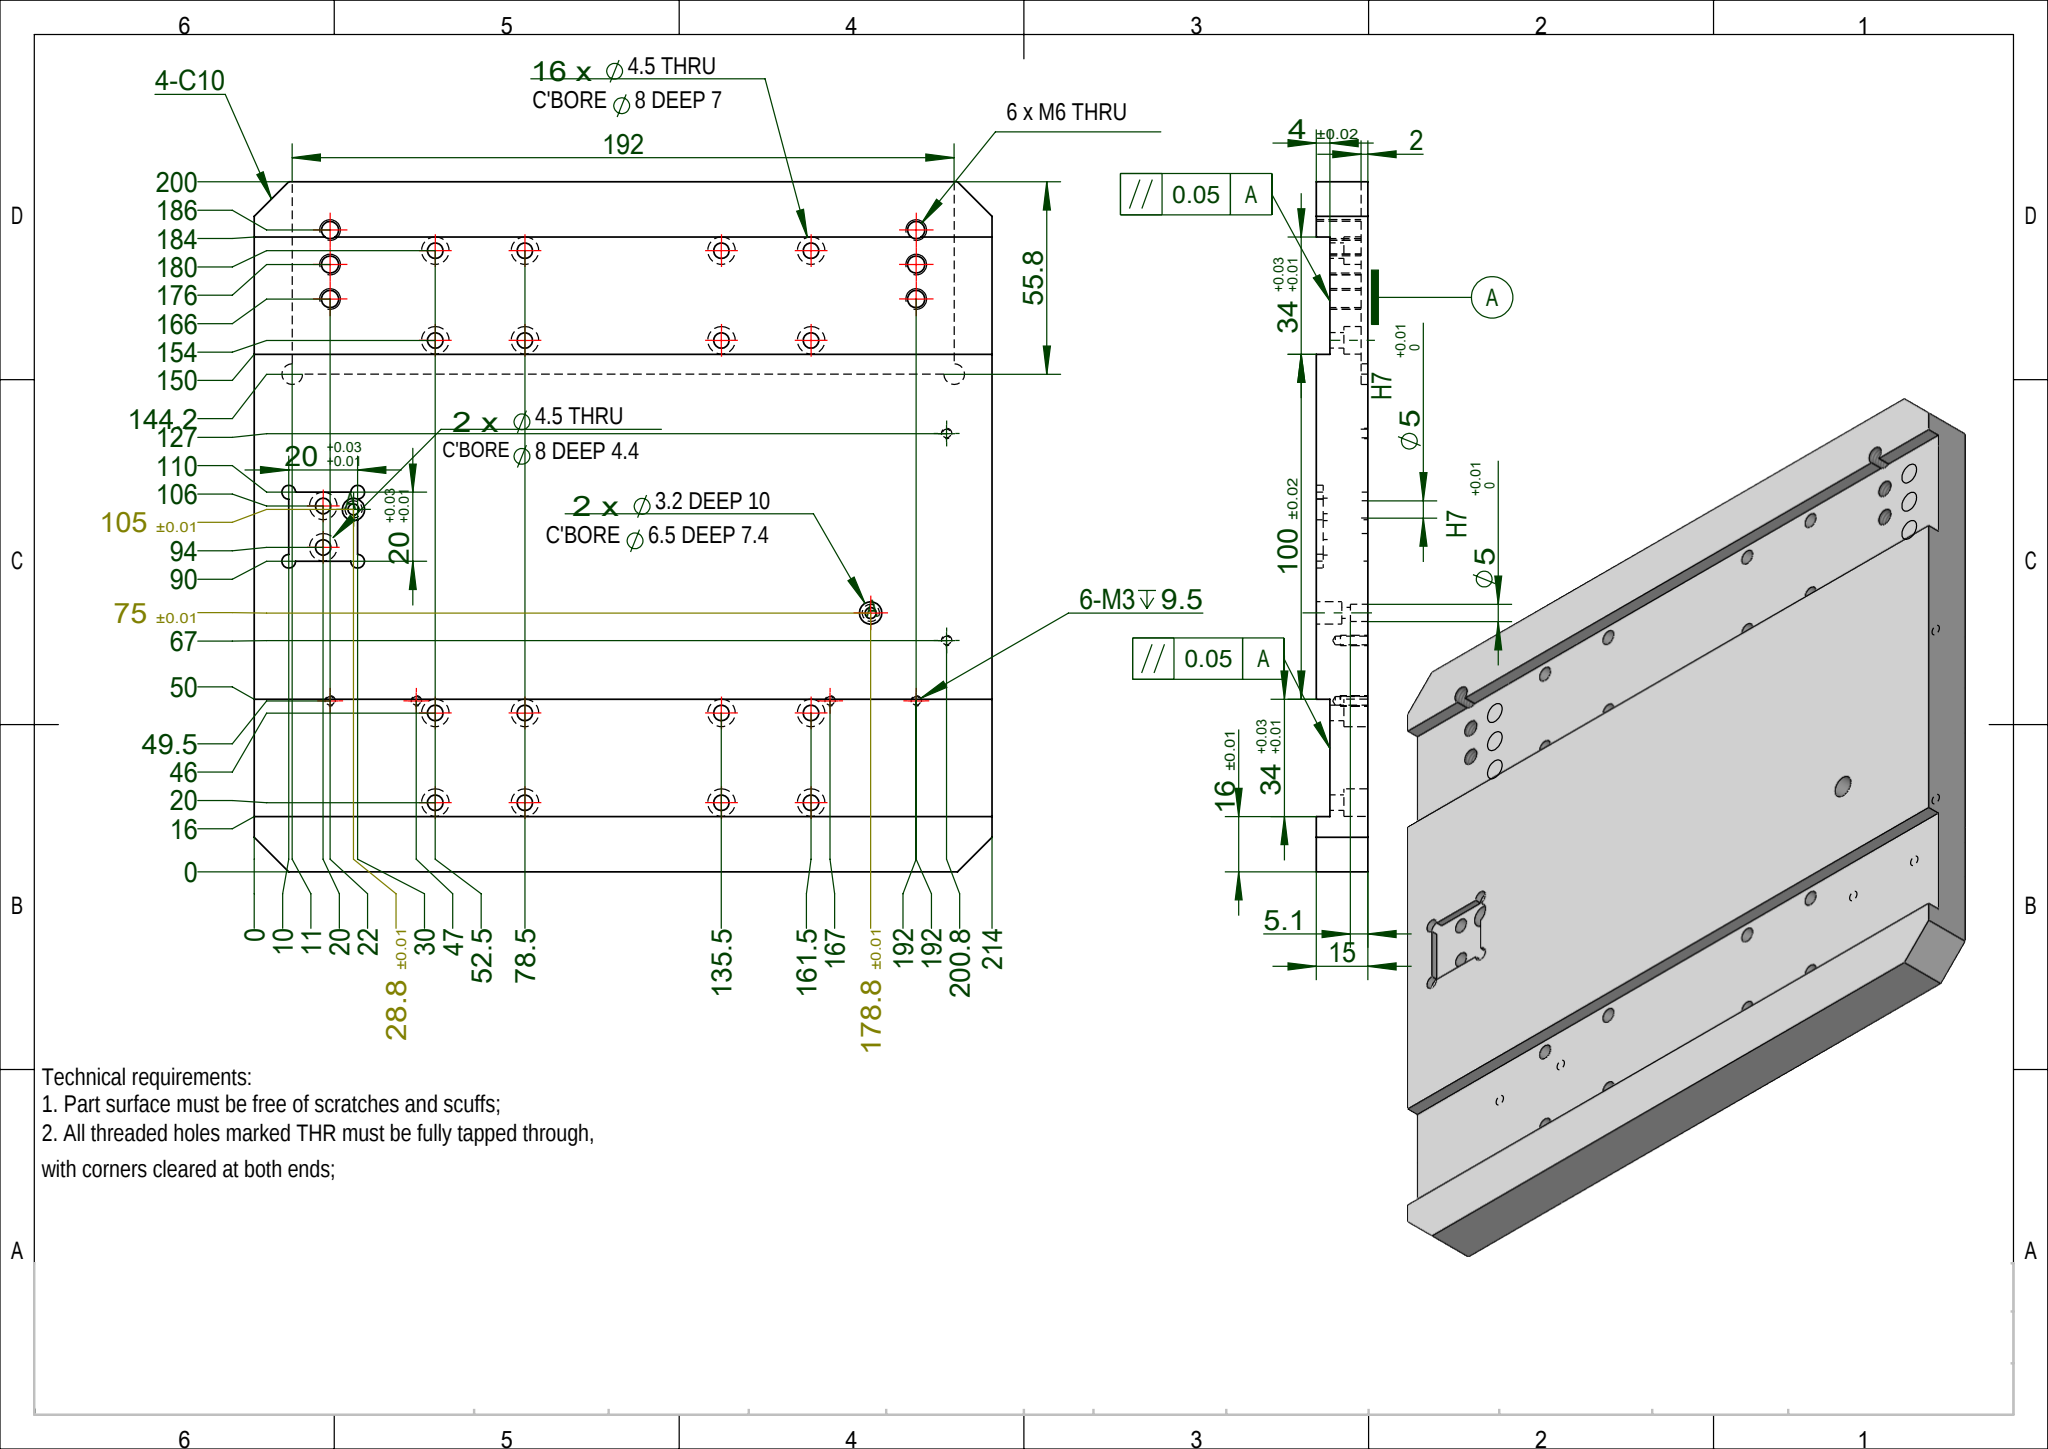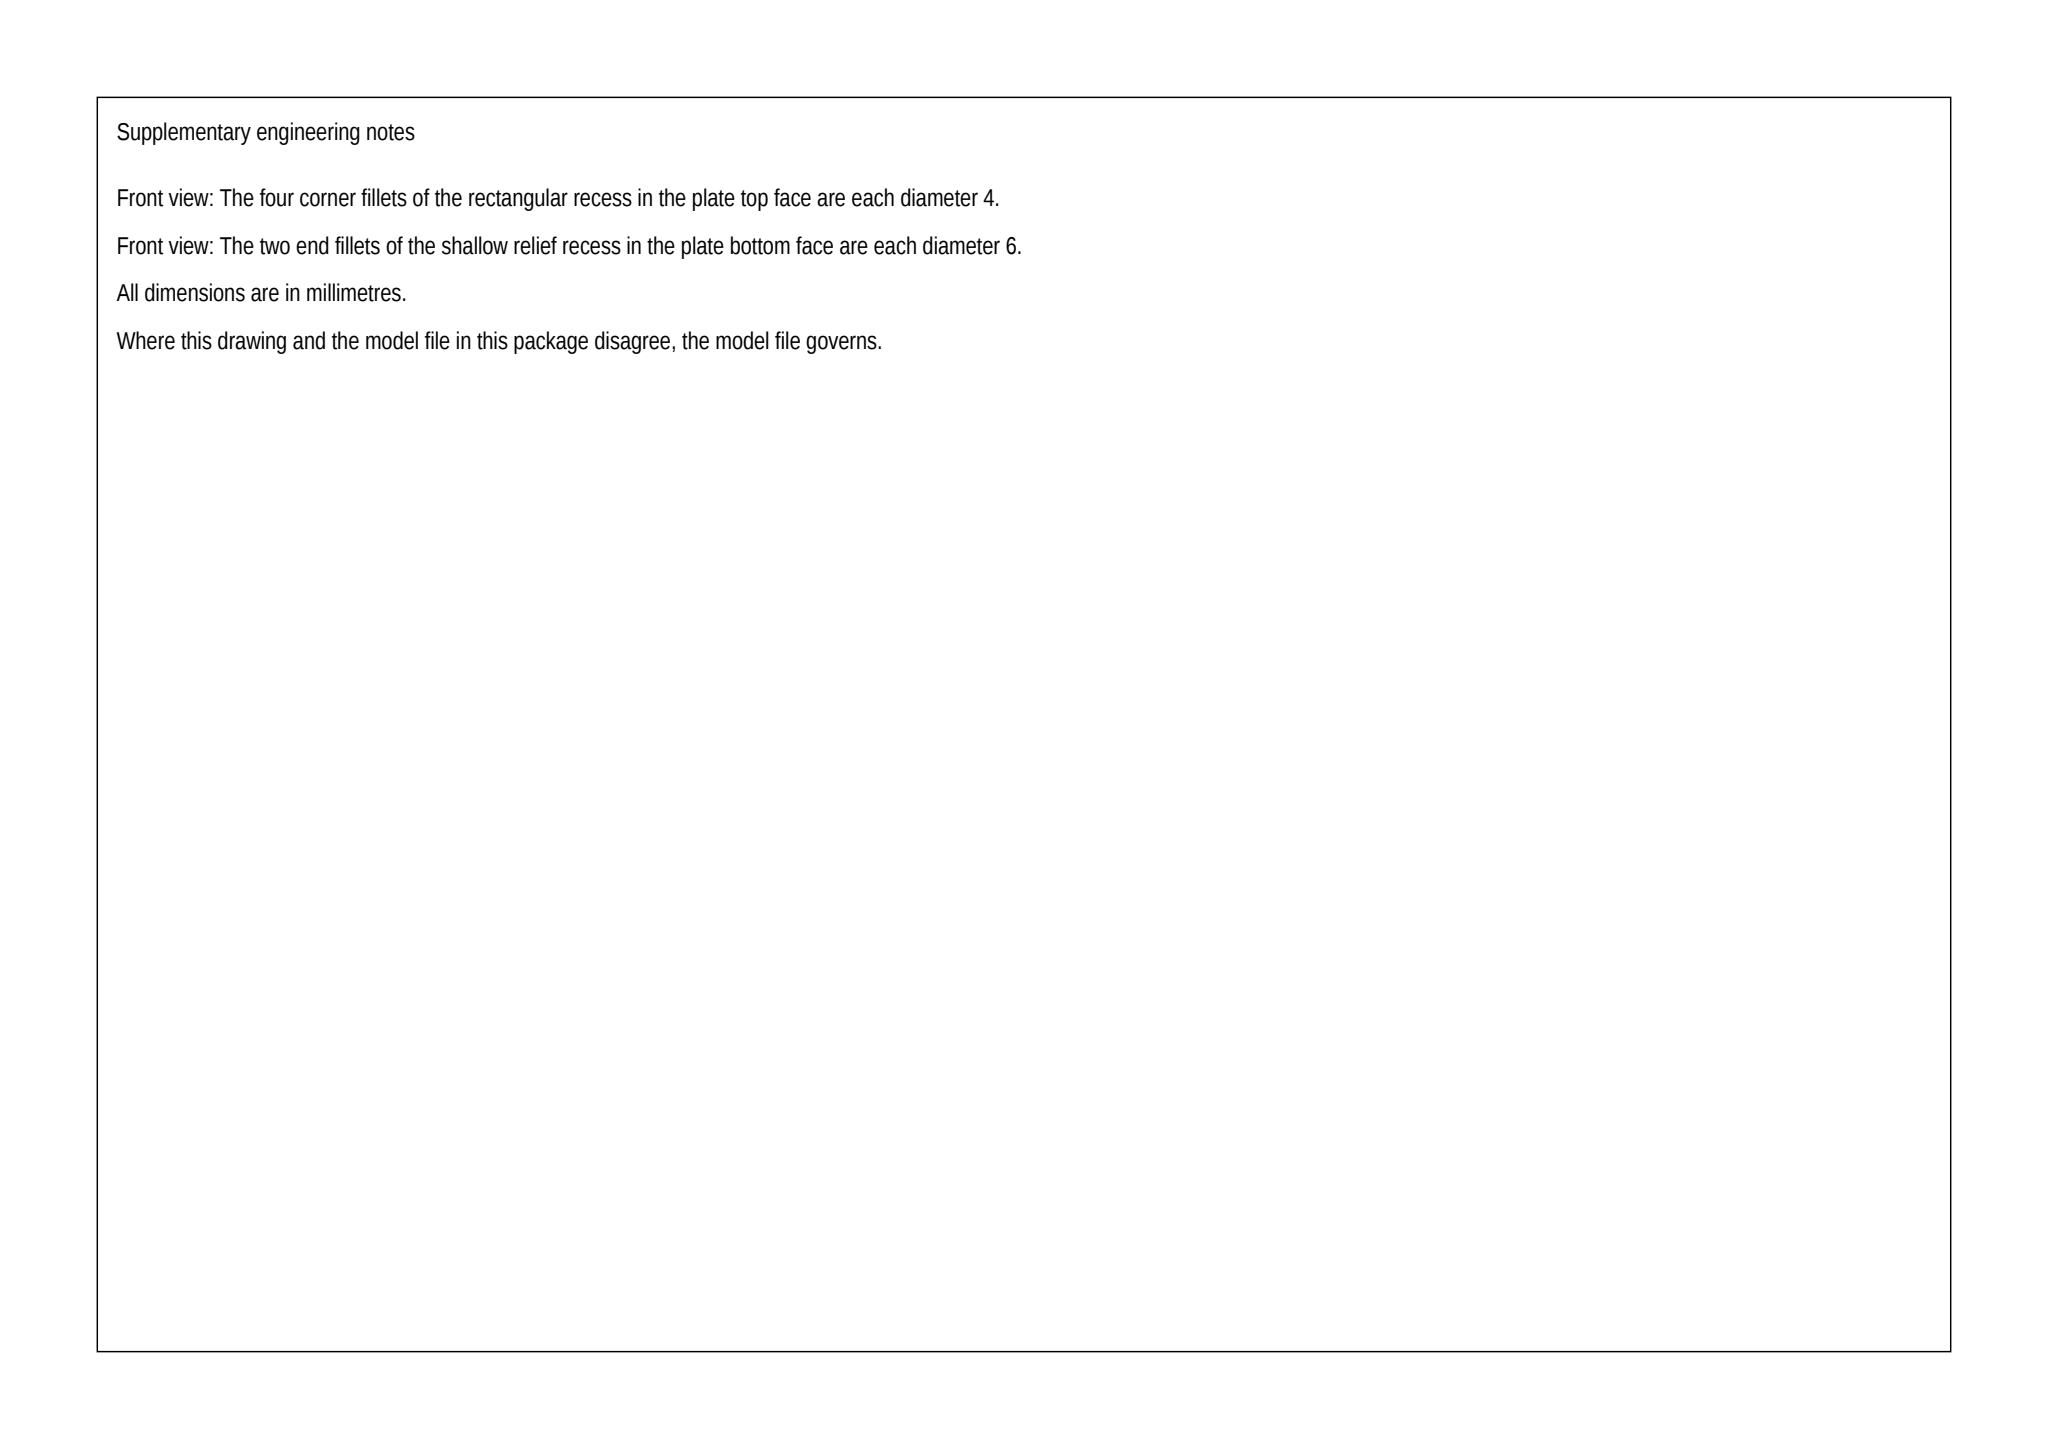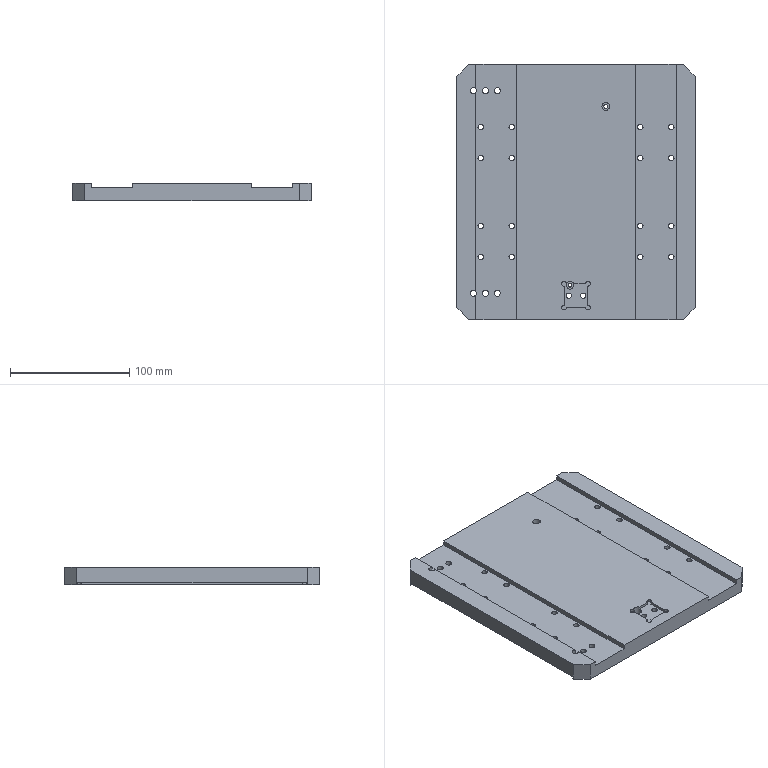Part | SolidWorks | mm | 1 solid | 179 faces | box 200 x 214 x 15 mm | volume 549666 mm3 | cylinder 116 | plane 51 | cone 12 | commonest cylinder face diameters 8 x36 4.5 x36 5 x16 2.5 x12 4 x6 6.5 x4 3.2 x4 6 x2
build123d program:
from build123d import *

# Parameters (mm, degrees)
SKETCH1_W                                       = 200
SKETCH1_H                                       = 214
BOSS_EXTRUDE1_DEPTH                             = 7.5
CHAMFER1_SIZE                                   = 10
M3_TAPPED_HOLE2_D                               = 2.5
M3_TAPPED_HOLE2_DEPTH                           = 9.5
M3_TAPPED_HOLE2_TIP                             = 0.7511
SIZE_MM_DOWEL_PIN_HOLE_1_D                      = 5
SIZE_MM_DOWEL_PIN_HOLE_1_DEPTH                  = 5.1
M4_HEX_SOCKET_HEAD_CAP_SCREW_CBORE1_D           = 4.5
M4_HEX_SOCKET_HEAD_CAP_SCREW_CBORE1_CBORE_D     = 8
M4_HEX_SOCKET_HEAD_CAP_SCREW_CBORE1_CBORE_DEPTH = 4.4
M4_HEX_SOCKET_HEAD_CAP_SCREW_CBORE2_D           = 4.5
M4_HEX_SOCKET_HEAD_CAP_SCREW_CBORE2_CBORE_D     = 8
M4_HEX_SOCKET_HEAD_CAP_SCREW_CBORE2_CBORE_DEPTH = 7
SKETCH28_W                                      = 20
SKETCH28_H                                      = 20
CUT_EXTRUDE3_DEPTH                              = 2
SKETCH29_R                                      = 2
CUT_EXTRUDE4_DEPTH                              = 2
SKETCH30_W                                      = 34
SKETCH30_H                                      = 214
CUT_EXTRUDE5_DEPTH                              = 4
SKETCH32_W                                      = 55.8
SKETCH32_H                                      = 192
CUT_EXTRUDE7_DEPTH                              = 2
SKETCH33_R                                      = 3
CUT_EXTRUDE8_DEPTH                              = 2
M6_TAPPED_HOLE1_D                               = 5
M3_HEX_SOCKET_HEAD_CAP_SCREW_CBORE1_D           = 3.2
M3_HEX_SOCKET_HEAD_CAP_SCREW_CBORE1_DEPTH       = 10
M3_HEX_SOCKET_HEAD_CAP_SCREW_CBORE1_CBORE_D     = 6.5
M3_HEX_SOCKET_HEAD_CAP_SCREW_CBORE1_CBORE_DEPTH = 7.4
M3_HEX_SOCKET_HEAD_CAP_SCREW_CBORE1_TIP         = 0.9614
M3_TAPPED_HOLE3_D                               = 2.5
M3_TAPPED_HOLE3_DEPTH                           = 9.5
M3_TAPPED_HOLE3_TIP                             = 0.7511


with BuildPart() as part:
    # Sketch1 → Boss-Extrude1 (new, symmetric)
    with BuildSketch(Plane.XY):
        Rectangle(SKETCH1_W, SKETCH1_H)
    extrude(amount=BOSS_EXTRUDE1_DEPTH, both=True)

    # Chamfer1
    chamfer1_edges = [part.edges().sort_by_distance(p)[0] for p in [
        (100, -107, 0),
        (-100, -107, 0),
        (-100, 107, 0),
        (100, 107, 0),
    ]]
    chamfer(chamfer1_edges, length=CHAMFER1_SIZE)

    # M3 Tapped Hole2
    with Locations(Plane(origin=(0, 0, -7.5), x_dir=(-1, 0, 0), z_dir=(0, 0, -1))):
        with Locations((-50.5, 85), (-50.5, 60), (-50.5, -60), (-50.5, -85)):
            Hole(M3_TAPPED_HOLE2_D / 2, depth=M3_TAPPED_HOLE2_DEPTH)
            with Locations((0, 0, -(M3_TAPPED_HOLE2_DEPTH + M3_TAPPED_HOLE2_TIP / 2))):  # 118° drill point
                Cone(0, M3_TAPPED_HOLE2_D / 2, M3_TAPPED_HOLE2_TIP, mode=Mode.SUBTRACT)

    # Size mm Dowel Pin Hole 1
    with Locations(Plane(origin=(0, 0, -7.5), x_dir=(-1, 0, 0), z_dir=(0, 0, -1))):
        with Locations((-25, 71.8), (5, -78.2)):
            Hole(SIZE_MM_DOWEL_PIN_HOLE_1_D / 2, depth=SIZE_MM_DOWEL_PIN_HOLE_1_DEPTH)

    # M4 Hex Socket Head Cap Screw CBORE1 (through all)
    with Locations(Plane(origin=(0, 0, -7.5), x_dir=(-1, 0, 0), z_dir=(0, 0, -1))):
        with Locations((-6, -87), (6, -87)):
            CounterBoreHole(M4_HEX_SOCKET_HEAD_CAP_SCREW_CBORE1_D / 2, M4_HEX_SOCKET_HEAD_CAP_SCREW_CBORE1_CBORE_D / 2, M4_HEX_SOCKET_HEAD_CAP_SCREW_CBORE1_CBORE_DEPTH)

    # M4 Hex Socket Head Cap Screw CBORE2 (through all)
    with Locations(Plane(origin=(0, 0, -7.5), x_dir=(-1, 0, 0), z_dir=(0, 0, -1))):
        with Locations((-80, 54.5), (-54, 54.5), (-54, 28.5), (-80, 28.5), (-80, -28.5), (-54, -28.5), (-54, -54.5), (-80, -54.5), (80, 54.5), (54, 54.5), (54, 28.5), (80, 28.5), (80, -28.5), (54, -28.5), (54, -54.5), (80, -54.5)):
            CounterBoreHole(M4_HEX_SOCKET_HEAD_CAP_SCREW_CBORE2_D / 2, M4_HEX_SOCKET_HEAD_CAP_SCREW_CBORE2_CBORE_D / 2, M4_HEX_SOCKET_HEAD_CAP_SCREW_CBORE2_CBORE_DEPTH)

    # Sketch28 → Cut-Extrude3 (cut)
    with BuildSketch(Plane.XY.offset(7.5)):
        with Locations((0, -87)):
            Rectangle(SKETCH28_W, SKETCH28_H)
    extrude(amount=-CUT_EXTRUDE3_DEPTH, mode=Mode.SUBTRACT)

    # Sketch29 → Cut-Extrude4 (cut)
    with BuildSketch(Plane.XY.offset(7.5)):
        with Locations((10, -97)):
            Circle(SKETCH29_R)
        with Locations((-10, -97)):
            Circle(SKETCH29_R)
        with Locations((-10, -77)):
            Circle(SKETCH29_R)
        with Locations((10, -77)):
            Circle(SKETCH29_R)
    extrude(amount=-CUT_EXTRUDE4_DEPTH, mode=Mode.SUBTRACT)

    # Sketch30 → Cut-Extrude5 (cut)
    with BuildSketch(Plane.XY.offset(7.5)):
        with Locations((67, 0)):
            Rectangle(SKETCH30_W, SKETCH30_H)
        with Locations((-67, 0)):
            Rectangle(SKETCH30_W, SKETCH30_H)
    extrude(amount=-CUT_EXTRUDE5_DEPTH, mode=Mode.SUBTRACT)

    # Sketch32 → Cut-Extrude7 (cut)
    with BuildSketch(Plane(origin=(0, 0, -7.5), x_dir=(-1, 0, 0), z_dir=(0, 0, -1))):
        with Locations((72.1, 0)):
            Rectangle(SKETCH32_W, SKETCH32_H)
    extrude(amount=-CUT_EXTRUDE7_DEPTH, mode=Mode.SUBTRACT)

    # Sketch33 → Cut-Extrude8 (cut)
    with BuildSketch(Plane(origin=(0, 0, -7.5), x_dir=(-1, 0, 0), z_dir=(0, 0, -1))):
        with Locations((44.2, -96)):
            Circle(SKETCH33_R)
        with Locations((44.2, 96)):
            Circle(SKETCH33_R)
    extrude(amount=-CUT_EXTRUDE8_DEPTH, mode=Mode.SUBTRACT)

    # M6 Tapped Hole1 (through all)
    with Locations(Plane(origin=(0, 0, -5.5), x_dir=(-1, 0, 0), z_dir=(0, 0, -1))):
        with Locations((66, -85), (66, 85), (76, -85), (86, -85), (76, 85), (86, 85)):
            Hole(M6_TAPPED_HOLE1_D / 2)

    # M3 Hex Socket Head Cap Screw CBORE1
    with Locations(Plane.XY.offset(7.5)):
        with Locations((-5, -78.2), (25, 71.8)):
            CounterBoreHole(M3_HEX_SOCKET_HEAD_CAP_SCREW_CBORE1_D / 2, M3_HEX_SOCKET_HEAD_CAP_SCREW_CBORE1_CBORE_D / 2, M3_HEX_SOCKET_HEAD_CAP_SCREW_CBORE1_CBORE_DEPTH, depth=M3_HEX_SOCKET_HEAD_CAP_SCREW_CBORE1_DEPTH)
            with Locations((0, 0, -(M3_HEX_SOCKET_HEAD_CAP_SCREW_CBORE1_DEPTH + M3_HEX_SOCKET_HEAD_CAP_SCREW_CBORE1_TIP / 2))):  # 118° drill point
                Cone(0, M3_HEX_SOCKET_HEAD_CAP_SCREW_CBORE1_D / 2, M3_HEX_SOCKET_HEAD_CAP_SCREW_CBORE1_TIP, mode=Mode.SUBTRACT)

    # M3 Tapped Hole3
    with Locations(Plane(origin=(0, 0, -7.5), x_dir=(-1, 0, 0), z_dir=(0, 0, -1))):
        with Locations((27, 93.8), (-33, 93.8)):
            Hole(M3_TAPPED_HOLE3_D / 2, depth=M3_TAPPED_HOLE3_DEPTH)
            with Locations((0, 0, -(M3_TAPPED_HOLE3_DEPTH + M3_TAPPED_HOLE3_TIP / 2))):  # 118° drill point
                Cone(0, M3_TAPPED_HOLE3_D / 2, M3_TAPPED_HOLE3_TIP, mode=Mode.SUBTRACT)


solid = part.part